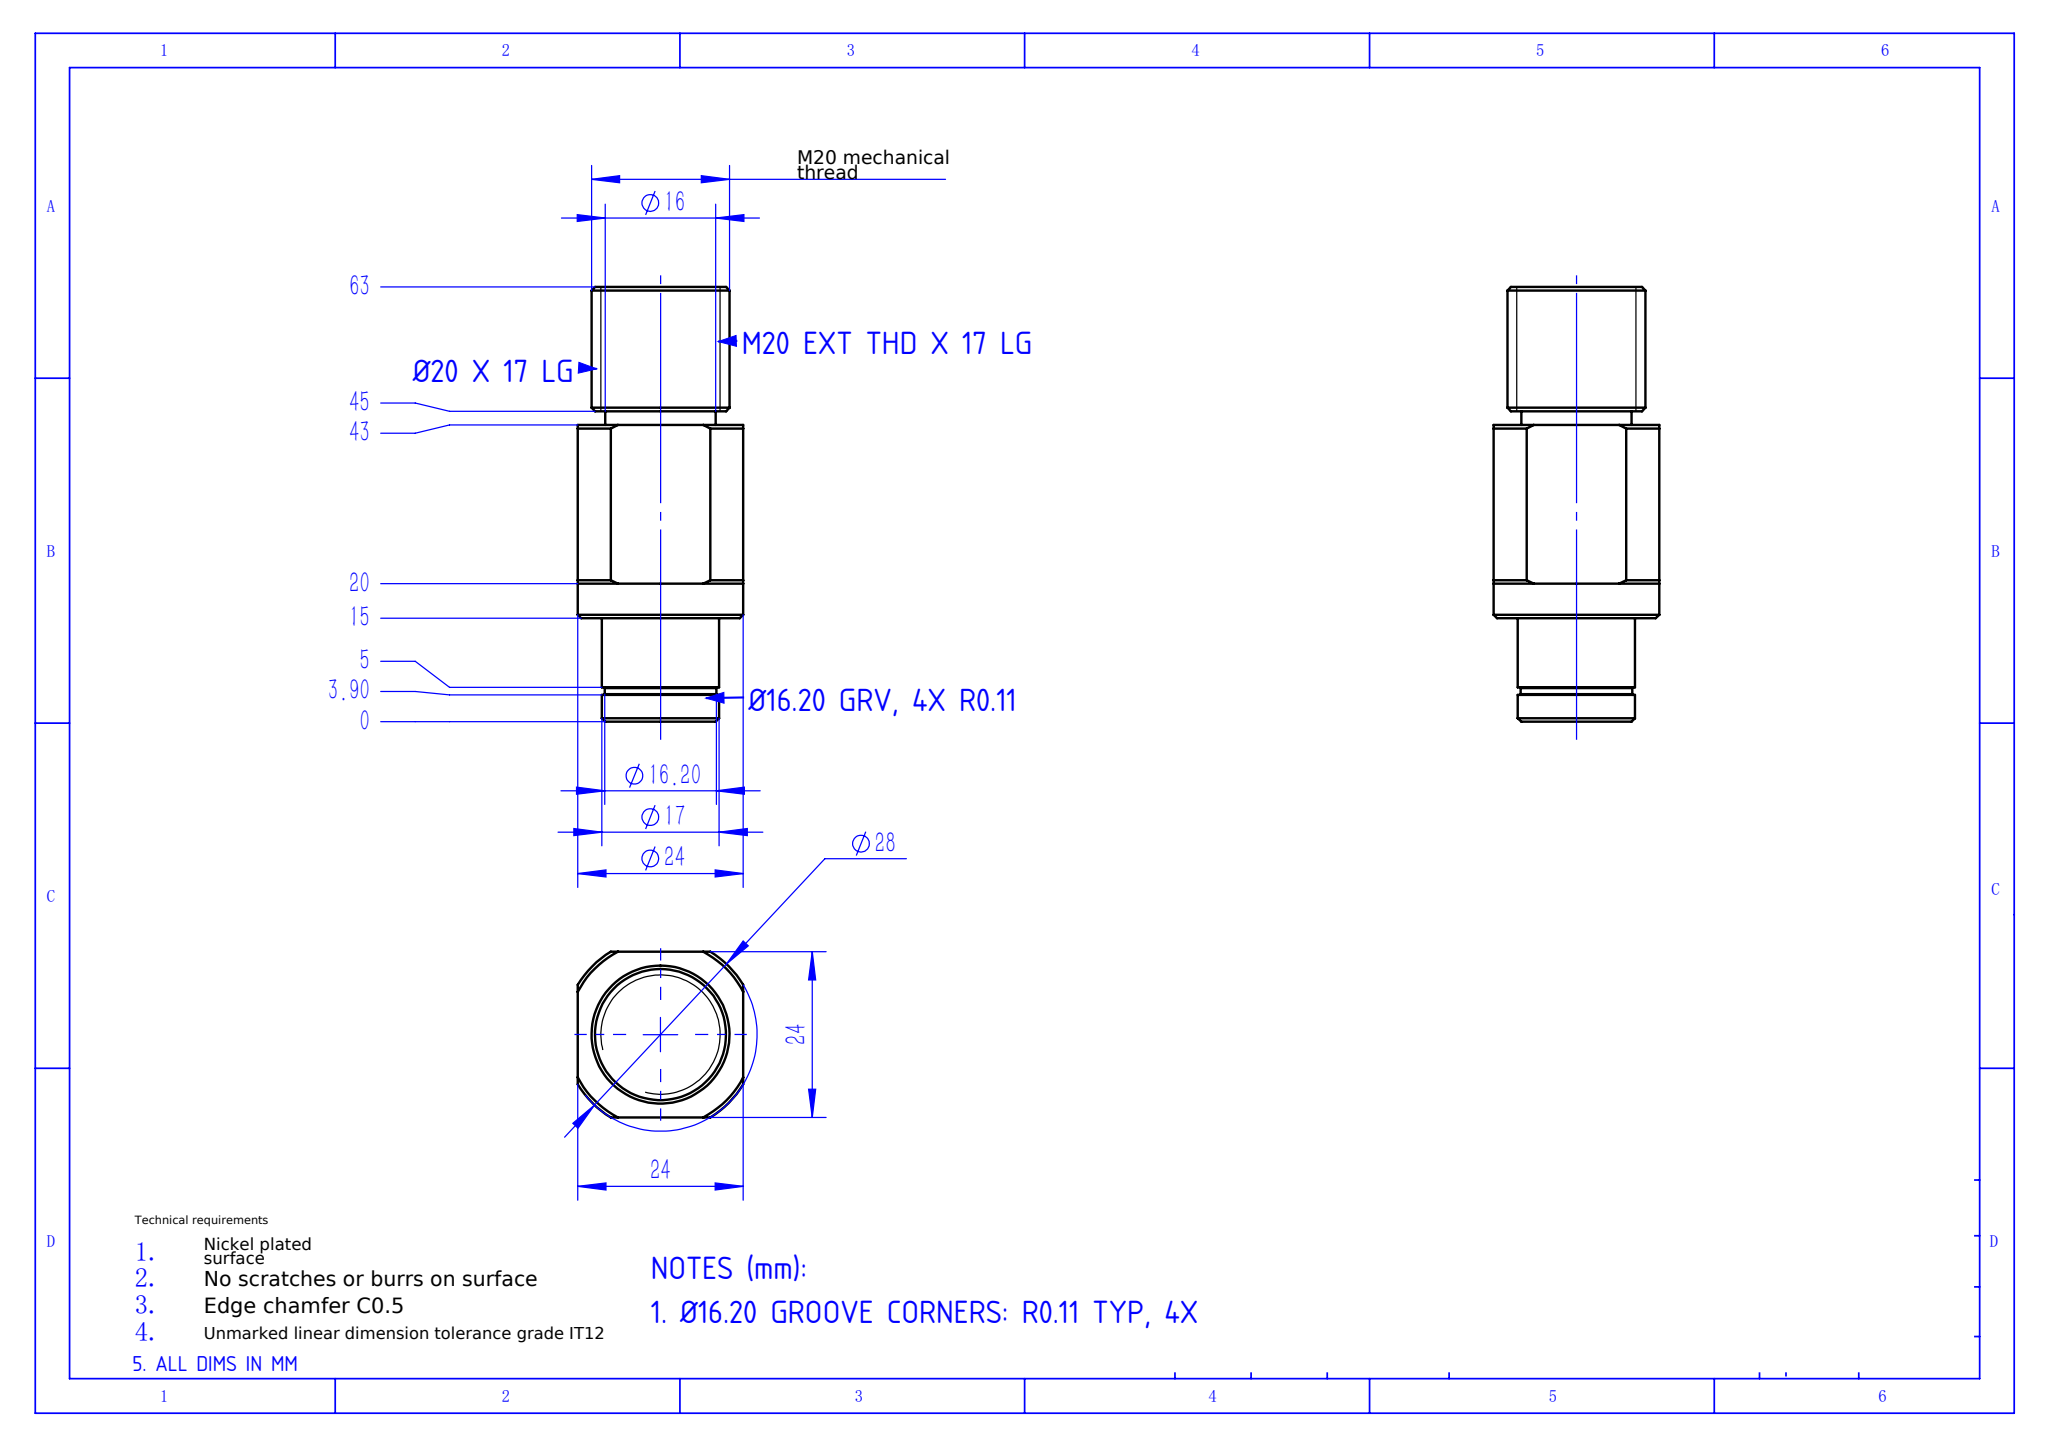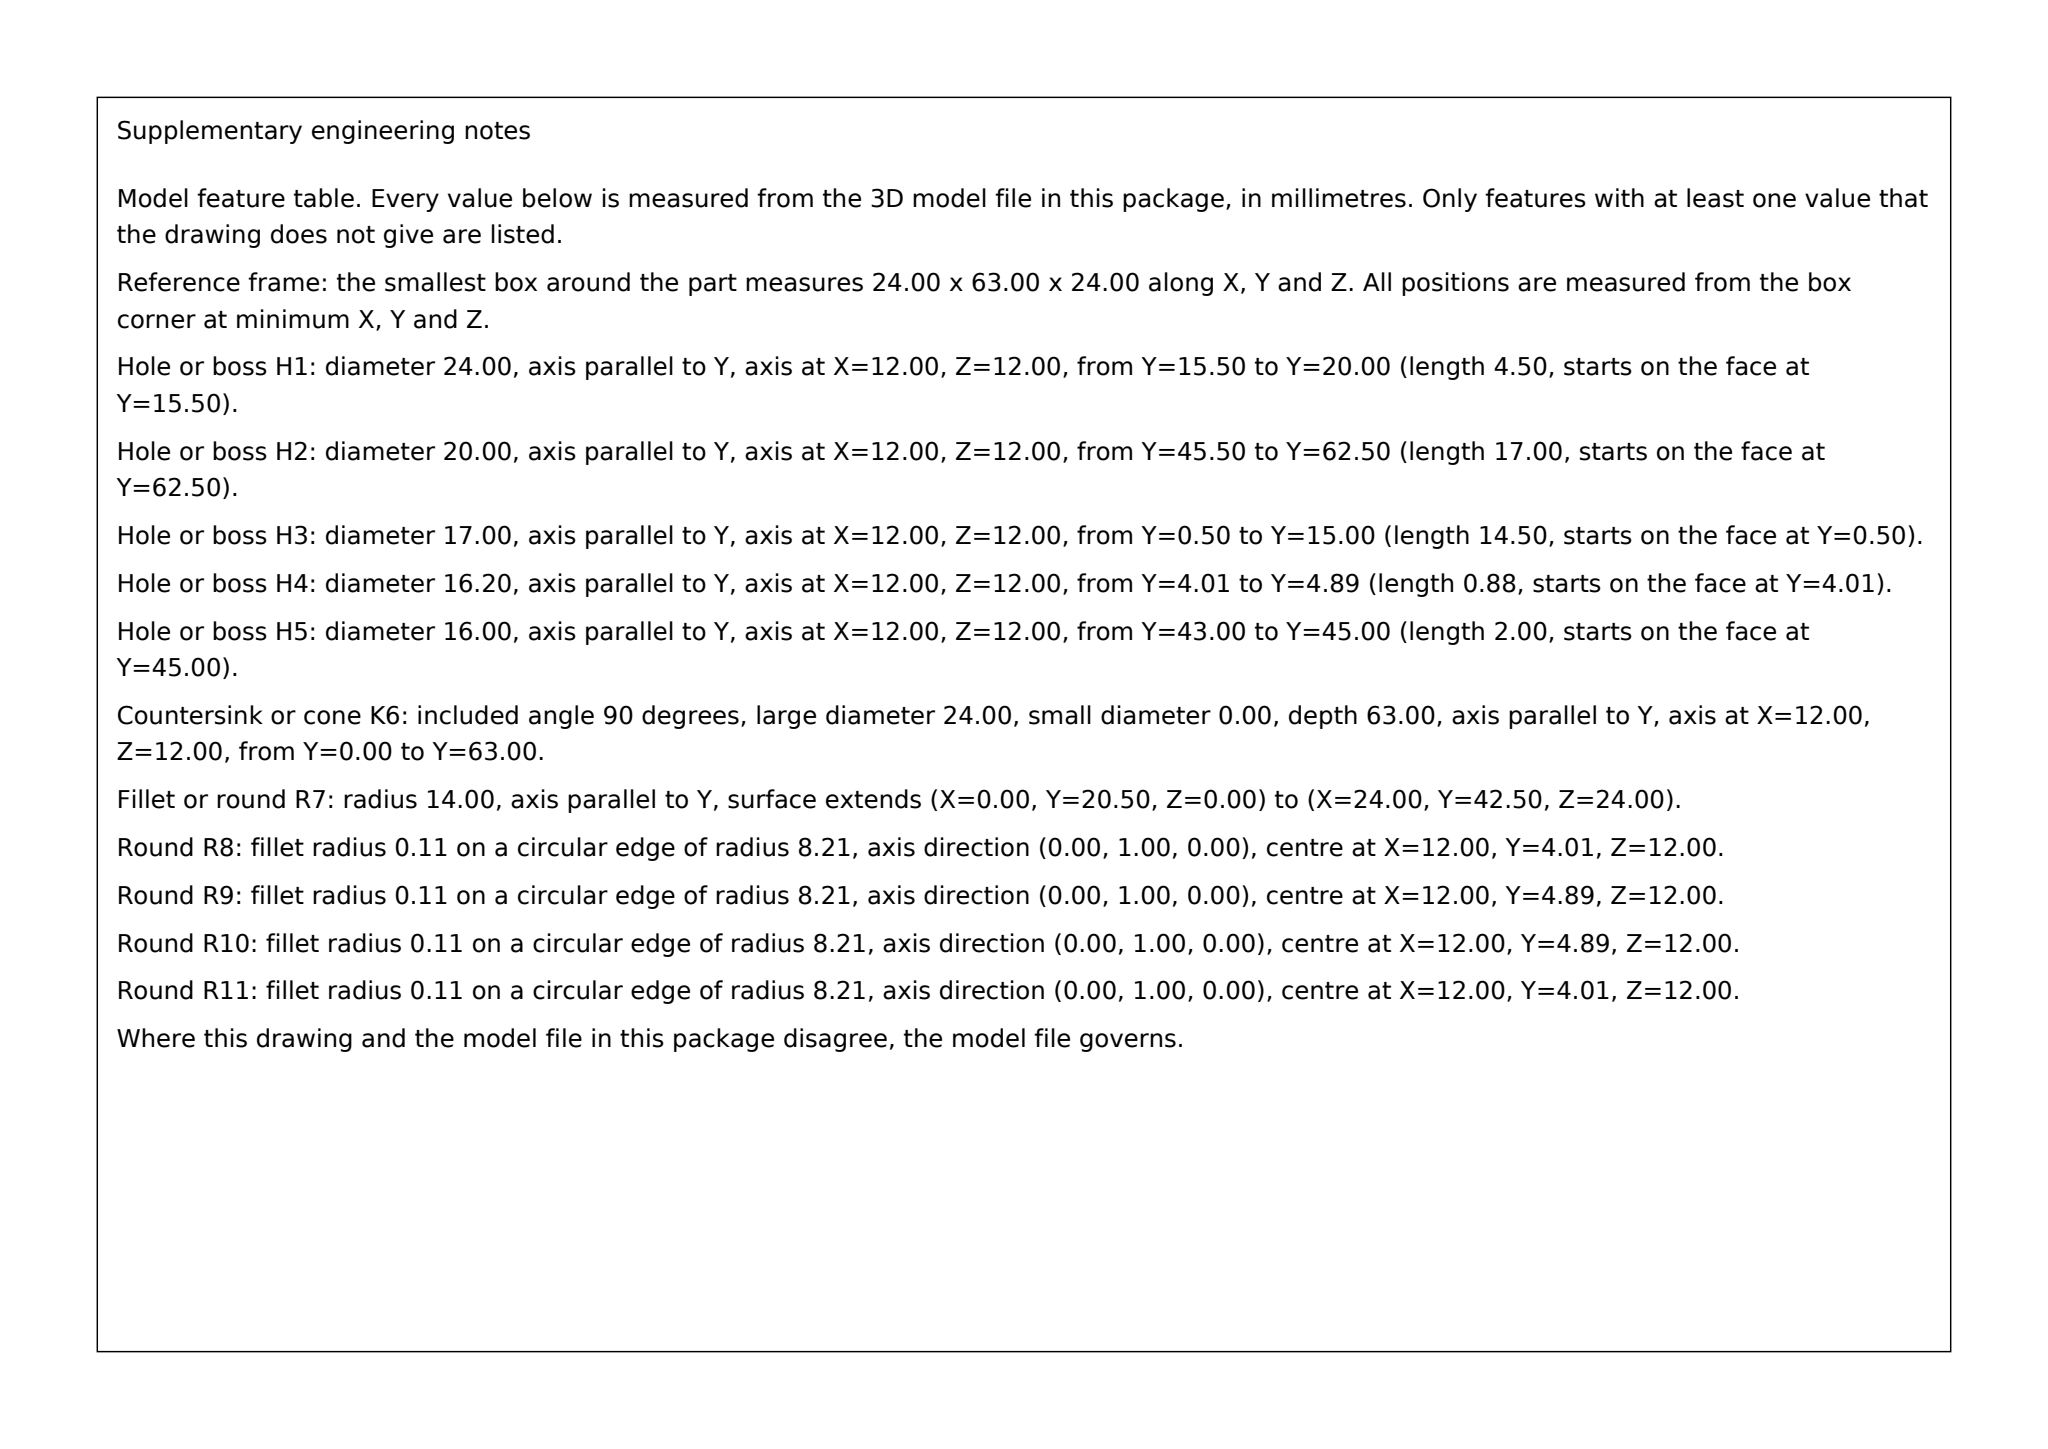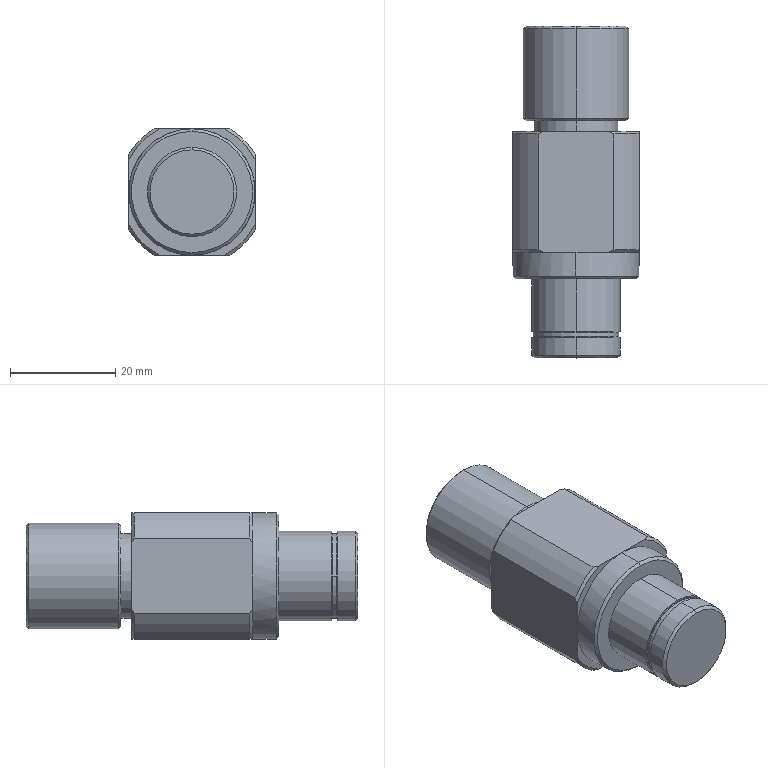Part | SolidWorks | mm | 1 solid | 51 faces | box 24 x 63 x 24 mm | volume 24029 mm3 | cone 16 | cylinder 16 | plane 15 | torus 4 | commonest cylinder face diameters 17 x4 28 x4 16.2 x2 24 x2 16 x2 20 x2
Drawing notes:
ALL DIMS IN MM | from the solid: STEP model units mm; bbox 24.889 x 63.0 x 24.889
Ø16.20 GROOVE CORNERS: R0.11 TYP, 4X | from the solid: tori [minor_r 0.11, major 8.21] x4 at Ø16.2 groove (y 4.0-4.9)
M20 EXT THD ON UPPER BOSS Ø20, 17 LG (45.5 TO 62.5) | from the solid: cylinder dia 20, axis y, from 45.5 to 62.5 = 17 LG
UPPER THD BOSS IS Ø20 X 17 LG, NOT Ø16 | from the solid: cylinder dia 20 from y45.5 to 62.5; Ø16 cyl only y43-45
NECK Ø16 X 2 LG, 43 TO 45, UNDER Ø20 THD BOSS | from the solid: cylinder dia 16, axis y, from 43.0 to 45.0 (2 LG)